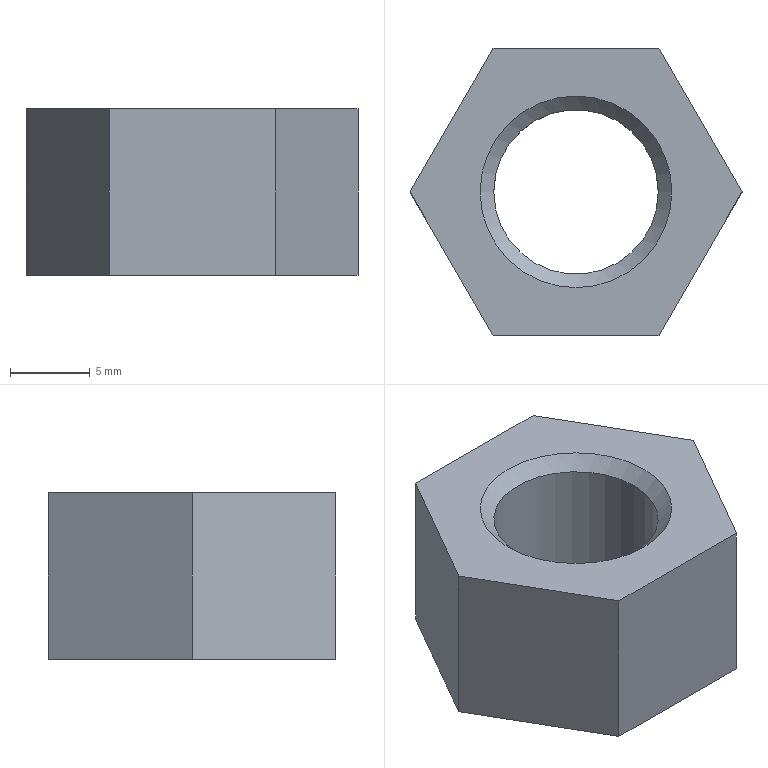Component | NX | 8_2 | 1 solid | 11 faces | box 20.78 x 18 x 10.4 mm | volume 2027 mm3 | plane 8 | cone 2 | cylinder 1 | commonest cylinder face diameters 10.3 x1
STEP:
#1=CARTESIAN_POINT('',(0.,0.,0.));
#2=DIRECTION('',(0.,0.,1.));
#3=DIRECTION('',(1.,0.,0.));
#4=AXIS2_PLACEMENT_3D('',#1,#2,#3);
#5=CARTESIAN_POINT('',(-19.608,30.,47.5));
#6=VERTEX_POINT('',#5);
#7=CARTESIAN_POINT('',(-24.804,39.,47.5));
#8=VERTEX_POINT('',#7);
#9=CARTESIAN_POINT('',(-19.608,30.,47.5));
#10=DIRECTION('',(-0.5,0.866,0.));
#11=VECTOR('',#10,1.);
#12=LINE('',#9,#11);
#13=CARTESIAN_POINT('',(-19.608,30.,57.9));
#14=DIRECTION('',(-0.866,-0.5,0.));
#15=DIRECTION('',(0.5,-0.866,0.));
#16=AXIS2_PLACEMENT_3D('',#13,#14,#15);
#17=PLANE('',#16);
#18=CARTESIAN_POINT('',(0.,-10.4));
#19=DIRECTION('',(-1.,0.));
#20=VECTOR('',#19,1.);
#21=LINE('',#18,#20);
#22=(GEOMETRIC_REPRESENTATION_CONTEXT(2)PARAMETRIC_REPRESENTATION_CONTEXT()REPRESENTATION_CONTEXT('',''));
#23=DEFINITIONAL_REPRESENTATION('',(#21),#22);
#24=PCURVE('',#17,#23);
#25=CARTESIAN_POINT('',(-30.,30.,47.5));
#26=DIRECTION('',(0.,0.,1.));
#27=DIRECTION('',(-1.,-0.00000005,0.));
#28=AXIS2_PLACEMENT_3D('',#25,#26,#27);
#29=PLANE('',#28);
#30=CARTESIAN_POINT('',(-10.392,0.));
#31=DIRECTION('',(0.5,-0.866));
#32=VECTOR('',#31,1.);
#33=LINE('',#30,#32);
#34=(GEOMETRIC_REPRESENTATION_CONTEXT(2)PARAMETRIC_REPRESENTATION_CONTEXT()REPRESENTATION_CONTEXT('',''));
#35=DEFINITIONAL_REPRESENTATION('',(#33),#34);
#36=PCURVE('',#29,#35);
#37=SURFACE_CURVE('',#12,(#24,#36),.PCURVE_S1.);
#38=EDGE_CURVE('',#6,#8,#37,.T.);
#39=ORIENTED_EDGE('',*,*,#38,.T.);
#40=CARTESIAN_POINT('',(-24.804,39.,57.9));
#41=VERTEX_POINT('',#40);
#42=CARTESIAN_POINT('',(-24.804,39.,57.9));
#43=DIRECTION('',(0.,0.,-1.));
#44=VECTOR('',#43,1.);
#45=LINE('',#42,#44);
#46=CARTESIAN_POINT('',(-10.392,0.));
#47=DIRECTION('',(0.,-1.));
#48=VECTOR('',#47,1.);
#49=LINE('',#46,#48);
#50=(GEOMETRIC_REPRESENTATION_CONTEXT(2)PARAMETRIC_REPRESENTATION_CONTEXT()REPRESENTATION_CONTEXT('',''));
#51=DEFINITIONAL_REPRESENTATION('',(#49),#50);
#52=PCURVE('',#17,#51);
#53=CARTESIAN_POINT('',(-24.804,39.,57.9));
#54=DIRECTION('',(0.00000005,-1.,0.));
#55=DIRECTION('',(1.,0.00000005,0.));
#56=AXIS2_PLACEMENT_3D('',#53,#54,#55);
#57=PLANE('',#56);
#58=CARTESIAN_POINT('',(0.,0.));
#59=DIRECTION('',(0.,-1.));
#60=VECTOR('',#59,1.);
#61=LINE('',#58,#60);
#62=(GEOMETRIC_REPRESENTATION_CONTEXT(2)PARAMETRIC_REPRESENTATION_CONTEXT()REPRESENTATION_CONTEXT('',''));
#63=DEFINITIONAL_REPRESENTATION('',(#61),#62);
#64=PCURVE('',#57,#63);
#65=SURFACE_CURVE('',#45,(#52,#64),.PCURVE_S1.);
#66=EDGE_CURVE('',#41,#8,#65,.T.);
#67=ORIENTED_EDGE('',*,*,#66,.F.);
#68=CARTESIAN_POINT('',(-19.608,30.,57.9));
#69=VERTEX_POINT('',#68);
#70=CARTESIAN_POINT('',(-19.608,30.,57.9));
#71=DIRECTION('',(-0.5,0.866,0.));
#72=VECTOR('',#71,1.);
#73=LINE('',#70,#72);
#74=CARTESIAN_POINT('',(0.,0.));
#75=DIRECTION('',(-1.,0.));
#76=VECTOR('',#75,1.);
#77=LINE('',#74,#76);
#78=(GEOMETRIC_REPRESENTATION_CONTEXT(2)PARAMETRIC_REPRESENTATION_CONTEXT()REPRESENTATION_CONTEXT('',''));
#79=DEFINITIONAL_REPRESENTATION('',(#77),#78);
#80=PCURVE('',#17,#79);
#81=CARTESIAN_POINT('',(-30.,30.,57.9));
#82=DIRECTION('',(0.,0.,1.));
#83=DIRECTION('',(-1.,-0.00000005,0.));
#84=AXIS2_PLACEMENT_3D('',#81,#82,#83);
#85=PLANE('',#84);
#86=CARTESIAN_POINT('',(-10.392,0.));
#87=DIRECTION('',(0.5,-0.866));
#88=VECTOR('',#87,1.);
#89=LINE('',#86,#88);
#90=(GEOMETRIC_REPRESENTATION_CONTEXT(2)PARAMETRIC_REPRESENTATION_CONTEXT()REPRESENTATION_CONTEXT('',''));
#91=DEFINITIONAL_REPRESENTATION('',(#89),#90);
#92=PCURVE('',#85,#91);
#93=SURFACE_CURVE('',#73,(#80,#92),.PCURVE_S1.);
#94=EDGE_CURVE('',#69,#41,#93,.T.);
#95=ORIENTED_EDGE('',*,*,#94,.F.);
#96=CARTESIAN_POINT('',(-19.608,30.,57.9));
#97=DIRECTION('',(0.,0.,-1.));
#98=VECTOR('',#97,1.);
#99=LINE('',#96,#98);
#100=CARTESIAN_POINT('',(0.,0.));
#101=DIRECTION('',(0.,-1.));
#102=VECTOR('',#101,1.);
#103=LINE('',#100,#102);
#104=(GEOMETRIC_REPRESENTATION_CONTEXT(2)PARAMETRIC_REPRESENTATION_CONTEXT()REPRESENTATION_CONTEXT('',''));
#105=DEFINITIONAL_REPRESENTATION('',(#103),#104);
#106=PCURVE('',#17,#105);
#107=CARTESIAN_POINT('',(-24.804,21.,57.9));
#108=DIRECTION('',(-0.866,0.5,0.));
#109=DIRECTION('',(-0.5,-0.866,0.));
#110=AXIS2_PLACEMENT_3D('',#107,#108,#109);
#111=PLANE('',#110);
#112=CARTESIAN_POINT('',(-10.392,0.));
#113=DIRECTION('',(0.,-1.));
#114=VECTOR('',#113,1.);
#115=LINE('',#112,#114);
#116=(GEOMETRIC_REPRESENTATION_CONTEXT(2)PARAMETRIC_REPRESENTATION_CONTEXT()REPRESENTATION_CONTEXT('',''));
#117=DEFINITIONAL_REPRESENTATION('',(#115),#116);
#118=PCURVE('',#111,#117);
#119=SURFACE_CURVE('',#99,(#106,#118),.PCURVE_S1.);
#120=EDGE_CURVE('',#69,#6,#119,.T.);
#121=ORIENTED_EDGE('',*,*,#120,.T.);
#122=EDGE_LOOP('',(#39,#67,#95,#121));
#123=FACE_BOUND('',#122,.T.);
#124=ADVANCED_FACE('',(#123),#17,.F.);
#125=CARTESIAN_POINT('',(-35.196,39.,47.5));
#126=VERTEX_POINT('',#125);
#127=CARTESIAN_POINT('',(-24.804,39.,47.5));
#128=DIRECTION('',(-1.,-0.00000005,0.));
#129=VECTOR('',#128,1.);
#130=LINE('',#127,#129);
#131=CARTESIAN_POINT('',(0.,-10.4));
#132=DIRECTION('',(-1.,0.));
#133=VECTOR('',#132,1.);
#134=LINE('',#131,#133);
#135=(GEOMETRIC_REPRESENTATION_CONTEXT(2)PARAMETRIC_REPRESENTATION_CONTEXT()REPRESENTATION_CONTEXT('',''));
#136=DEFINITIONAL_REPRESENTATION('',(#134),#135);
#137=PCURVE('',#57,#136);
#138=CARTESIAN_POINT('',(-5.196,-9.));
#139=DIRECTION('',(1.,-0.));
#140=VECTOR('',#139,1.);
#141=LINE('',#138,#140);
#142=(GEOMETRIC_REPRESENTATION_CONTEXT(2)PARAMETRIC_REPRESENTATION_CONTEXT()REPRESENTATION_CONTEXT('',''));
#143=DEFINITIONAL_REPRESENTATION('',(#141),#142);
#144=PCURVE('',#29,#143);
#145=SURFACE_CURVE('',#130,(#137,#144),.PCURVE_S1.);
#146=EDGE_CURVE('',#8,#126,#145,.T.);
#147=ORIENTED_EDGE('',*,*,#146,.T.);
#148=CARTESIAN_POINT('',(-35.196,39.,57.9));
#149=VERTEX_POINT('',#148);
#150=CARTESIAN_POINT('',(-35.196,39.,57.9));
#151=DIRECTION('',(0.,0.,-1.));
#152=VECTOR('',#151,1.);
#153=LINE('',#150,#152);
#154=CARTESIAN_POINT('',(-10.392,0.));
#155=DIRECTION('',(0.,-1.));
#156=VECTOR('',#155,1.);
#157=LINE('',#154,#156);
#158=(GEOMETRIC_REPRESENTATION_CONTEXT(2)PARAMETRIC_REPRESENTATION_CONTEXT()REPRESENTATION_CONTEXT('',''));
#159=DEFINITIONAL_REPRESENTATION('',(#157),#158);
#160=PCURVE('',#57,#159);
#161=CARTESIAN_POINT('',(-35.196,39.,57.9));
#162=DIRECTION('',(0.866,-0.5,0.));
#163=DIRECTION('',(0.5,0.866,0.));
#164=AXIS2_PLACEMENT_3D('',#161,#162,#163);
#165=PLANE('',#164);
#166=CARTESIAN_POINT('',(0.,0.));
#167=DIRECTION('',(0.,-1.));
#168=VECTOR('',#167,1.);
#169=LINE('',#166,#168);
#170=(GEOMETRIC_REPRESENTATION_CONTEXT(2)PARAMETRIC_REPRESENTATION_CONTEXT()REPRESENTATION_CONTEXT('',''));
#171=DEFINITIONAL_REPRESENTATION('',(#169),#170);
#172=PCURVE('',#165,#171);
#173=SURFACE_CURVE('',#153,(#160,#172),.PCURVE_S1.);
#174=EDGE_CURVE('',#149,#126,#173,.T.);
#175=ORIENTED_EDGE('',*,*,#174,.F.);
#176=CARTESIAN_POINT('',(-24.804,39.,57.9));
#177=DIRECTION('',(-1.,-0.00000005,0.));
#178=VECTOR('',#177,1.);
#179=LINE('',#176,#178);
#180=CARTESIAN_POINT('',(0.,0.));
#181=DIRECTION('',(-1.,0.));
#182=VECTOR('',#181,1.);
#183=LINE('',#180,#182);
#184=(GEOMETRIC_REPRESENTATION_CONTEXT(2)PARAMETRIC_REPRESENTATION_CONTEXT()REPRESENTATION_CONTEXT('',''));
#185=DEFINITIONAL_REPRESENTATION('',(#183),#184);
#186=PCURVE('',#57,#185);
#187=CARTESIAN_POINT('',(-5.196,-9.));
#188=DIRECTION('',(1.,-0.));
#189=VECTOR('',#188,1.);
#190=LINE('',#187,#189);
#191=(GEOMETRIC_REPRESENTATION_CONTEXT(2)PARAMETRIC_REPRESENTATION_CONTEXT()REPRESENTATION_CONTEXT('',''));
#192=DEFINITIONAL_REPRESENTATION('',(#190),#191);
#193=PCURVE('',#85,#192);
#194=SURFACE_CURVE('',#179,(#186,#193),.PCURVE_S1.);
#195=EDGE_CURVE('',#41,#149,#194,.T.);
#196=ORIENTED_EDGE('',*,*,#195,.F.);
#197=ORIENTED_EDGE('',*,*,#66,.T.);
#198=EDGE_LOOP('',(#147,#175,#196,#197));
#199=FACE_BOUND('',#198,.T.);
#200=ADVANCED_FACE('',(#199),#57,.F.);
#201=CARTESIAN_POINT('',(-40.392,30.,47.5));
#202=VERTEX_POINT('',#201);
#203=CARTESIAN_POINT('',(-35.196,39.,47.5));
#204=DIRECTION('',(-0.5,-0.866,0.));
#205=VECTOR('',#204,1.);
#206=LINE('',#203,#205);
#207=CARTESIAN_POINT('',(0.,-10.4));
#208=DIRECTION('',(-1.,0.));
#209=VECTOR('',#208,1.);
#210=LINE('',#207,#209);
#211=(GEOMETRIC_REPRESENTATION_CONTEXT(2)PARAMETRIC_REPRESENTATION_CONTEXT()REPRESENTATION_CONTEXT('',''));
#212=DEFINITIONAL_REPRESENTATION('',(#210),#211);
#213=PCURVE('',#165,#212);
#214=CARTESIAN_POINT('',(5.196,-9.));
#215=DIRECTION('',(0.5,0.866));
#216=VECTOR('',#215,1.);
#217=LINE('',#214,#216);
#218=(GEOMETRIC_REPRESENTATION_CONTEXT(2)PARAMETRIC_REPRESENTATION_CONTEXT()REPRESENTATION_CONTEXT('',''));
#219=DEFINITIONAL_REPRESENTATION('',(#217),#218);
#220=PCURVE('',#29,#219);
#221=SURFACE_CURVE('',#206,(#213,#220),.PCURVE_S1.);
#222=EDGE_CURVE('',#126,#202,#221,.T.);
#223=ORIENTED_EDGE('',*,*,#222,.T.);
#224=CARTESIAN_POINT('',(-40.392,30.,57.9));
#225=VERTEX_POINT('',#224);
#226=CARTESIAN_POINT('',(-40.392,30.,57.9));
#227=DIRECTION('',(0.,0.,-1.));
#228=VECTOR('',#227,1.);
#229=LINE('',#226,#228);
#230=CARTESIAN_POINT('',(-10.392,0.));
#231=DIRECTION('',(0.,-1.));
#232=VECTOR('',#231,1.);
#233=LINE('',#230,#232);
#234=(GEOMETRIC_REPRESENTATION_CONTEXT(2)PARAMETRIC_REPRESENTATION_CONTEXT()REPRESENTATION_CONTEXT('',''));
#235=DEFINITIONAL_REPRESENTATION('',(#233),#234);
#236=PCURVE('',#165,#235);
#237=CARTESIAN_POINT('',(-40.392,30.,57.9));
#238=DIRECTION('',(0.866,0.5,0.));
#239=DIRECTION('',(-0.5,0.866,0.));
#240=AXIS2_PLACEMENT_3D('',#237,#238,#239);
#241=PLANE('',#240);
#242=CARTESIAN_POINT('',(0.,0.));
#243=DIRECTION('',(0.,-1.));
#244=VECTOR('',#243,1.);
#245=LINE('',#242,#244);
#246=(GEOMETRIC_REPRESENTATION_CONTEXT(2)PARAMETRIC_REPRESENTATION_CONTEXT()REPRESENTATION_CONTEXT('',''));
#247=DEFINITIONAL_REPRESENTATION('',(#245),#246);
#248=PCURVE('',#241,#247);
#249=SURFACE_CURVE('',#229,(#236,#248),.PCURVE_S1.);
#250=EDGE_CURVE('',#225,#202,#249,.T.);
#251=ORIENTED_EDGE('',*,*,#250,.F.);
#252=CARTESIAN_POINT('',(-35.196,39.,57.9));
#253=DIRECTION('',(-0.5,-0.866,0.));
#254=VECTOR('',#253,1.);
#255=LINE('',#252,#254);
#256=CARTESIAN_POINT('',(0.,0.));
#257=DIRECTION('',(-1.,0.));
#258=VECTOR('',#257,1.);
#259=LINE('',#256,#258);
#260=(GEOMETRIC_REPRESENTATION_CONTEXT(2)PARAMETRIC_REPRESENTATION_CONTEXT()REPRESENTATION_CONTEXT('',''));
#261=DEFINITIONAL_REPRESENTATION('',(#259),#260);
#262=PCURVE('',#165,#261);
#263=CARTESIAN_POINT('',(5.196,-9.));
#264=DIRECTION('',(0.5,0.866));
#265=VECTOR('',#264,1.);
#266=LINE('',#263,#265);
#267=(GEOMETRIC_REPRESENTATION_CONTEXT(2)PARAMETRIC_REPRESENTATION_CONTEXT()REPRESENTATION_CONTEXT('',''));
#268=DEFINITIONAL_REPRESENTATION('',(#266),#267);
#269=PCURVE('',#85,#268);
#270=SURFACE_CURVE('',#255,(#262,#269),.PCURVE_S1.);
#271=EDGE_CURVE('',#149,#225,#270,.T.);
#272=ORIENTED_EDGE('',*,*,#271,.F.);
#273=ORIENTED_EDGE('',*,*,#174,.T.);
#274=EDGE_LOOP('',(#223,#251,#272,#273));
#275=FACE_BOUND('',#274,.T.);
#276=ADVANCED_FACE('',(#275),#165,.F.);
#277=CARTESIAN_POINT('',(-35.196,21.,47.5));
#278=VERTEX_POINT('',#277);
#279=CARTESIAN_POINT('',(-40.392,30.,47.5));
#280=DIRECTION('',(0.5,-0.866,0.));
#281=VECTOR('',#280,1.);
#282=LINE('',#279,#281);
#283=CARTESIAN_POINT('',(0.,-10.4));
#284=DIRECTION('',(-1.,0.));
#285=VECTOR('',#284,1.);
#286=LINE('',#283,#285);
#287=(GEOMETRIC_REPRESENTATION_CONTEXT(2)PARAMETRIC_REPRESENTATION_CONTEXT()REPRESENTATION_CONTEXT('',''));
#288=DEFINITIONAL_REPRESENTATION('',(#286),#287);
#289=PCURVE('',#241,#288);
#290=CARTESIAN_POINT('',(10.392,-0.));
#291=DIRECTION('',(-0.5,0.866));
#292=VECTOR('',#291,1.);
#293=LINE('',#290,#292);
#294=(GEOMETRIC_REPRESENTATION_CONTEXT(2)PARAMETRIC_REPRESENTATION_CONTEXT()REPRESENTATION_CONTEXT('',''));
#295=DEFINITIONAL_REPRESENTATION('',(#293),#294);
#296=PCURVE('',#29,#295);
#297=SURFACE_CURVE('',#282,(#289,#296),.PCURVE_S1.);
#298=EDGE_CURVE('',#202,#278,#297,.T.);
#299=ORIENTED_EDGE('',*,*,#298,.T.);
#300=CARTESIAN_POINT('',(-35.196,21.,57.9));
#301=VERTEX_POINT('',#300);
#302=CARTESIAN_POINT('',(-35.196,21.,57.9));
#303=DIRECTION('',(0.,0.,-1.));
#304=VECTOR('',#303,1.);
#305=LINE('',#302,#304);
#306=CARTESIAN_POINT('',(-10.392,0.));
#307=DIRECTION('',(0.,-1.));
#308=VECTOR('',#307,1.);
#309=LINE('',#306,#308);
#310=(GEOMETRIC_REPRESENTATION_CONTEXT(2)PARAMETRIC_REPRESENTATION_CONTEXT()REPRESENTATION_CONTEXT('',''));
#311=DEFINITIONAL_REPRESENTATION('',(#309),#310);
#312=PCURVE('',#241,#311);
#313=CARTESIAN_POINT('',(-35.196,21.,57.9));
#314=DIRECTION('',(-0.00000005,1.,0.));
#315=DIRECTION('',(-1.,-0.00000005,0.));
#316=AXIS2_PLACEMENT_3D('',#313,#314,#315);
#317=PLANE('',#316);
#318=CARTESIAN_POINT('',(0.,0.));
#319=DIRECTION('',(0.,-1.));
#320=VECTOR('',#319,1.);
#321=LINE('',#318,#320);
#322=(GEOMETRIC_REPRESENTATION_CONTEXT(2)PARAMETRIC_REPRESENTATION_CONTEXT()REPRESENTATION_CONTEXT('',''));
#323=DEFINITIONAL_REPRESENTATION('',(#321),#322);
#324=PCURVE('',#317,#323);
#325=SURFACE_CURVE('',#305,(#312,#324),.PCURVE_S1.);
#326=EDGE_CURVE('',#301,#278,#325,.T.);
#327=ORIENTED_EDGE('',*,*,#326,.F.);
#328=CARTESIAN_POINT('',(-40.392,30.,57.9));
#329=DIRECTION('',(0.5,-0.866,0.));
#330=VECTOR('',#329,1.);
#331=LINE('',#328,#330);
#332=CARTESIAN_POINT('',(0.,0.));
#333=DIRECTION('',(-1.,0.));
#334=VECTOR('',#333,1.);
#335=LINE('',#332,#334);
#336=(GEOMETRIC_REPRESENTATION_CONTEXT(2)PARAMETRIC_REPRESENTATION_CONTEXT()REPRESENTATION_CONTEXT('',''));
#337=DEFINITIONAL_REPRESENTATION('',(#335),#336);
#338=PCURVE('',#241,#337);
#339=CARTESIAN_POINT('',(10.392,-0.));
#340=DIRECTION('',(-0.5,0.866));
#341=VECTOR('',#340,1.);
#342=LINE('',#339,#341);
#343=(GEOMETRIC_REPRESENTATION_CONTEXT(2)PARAMETRIC_REPRESENTATION_CONTEXT()REPRESENTATION_CONTEXT('',''));
#344=DEFINITIONAL_REPRESENTATION('',(#342),#343);
#345=PCURVE('',#85,#344);
#346=SURFACE_CURVE('',#331,(#338,#345),.PCURVE_S1.);
#347=EDGE_CURVE('',#225,#301,#346,.T.);
#348=ORIENTED_EDGE('',*,*,#347,.F.);
#349=ORIENTED_EDGE('',*,*,#250,.T.);
#350=EDGE_LOOP('',(#299,#327,#348,#349));
#351=FACE_BOUND('',#350,.T.);
#352=ADVANCED_FACE('',(#351),#241,.F.);
#353=CARTESIAN_POINT('',(-24.804,21.,47.5));
#354=VERTEX_POINT('',#353);
#355=CARTESIAN_POINT('',(-35.196,21.,47.5));
#356=DIRECTION('',(1.,0.00000005,0.));
#357=VECTOR('',#356,1.);
#358=LINE('',#355,#357);
#359=CARTESIAN_POINT('',(0.,-10.4));
#360=DIRECTION('',(-1.,0.));
#361=VECTOR('',#360,1.);
#362=LINE('',#359,#361);
#363=(GEOMETRIC_REPRESENTATION_CONTEXT(2)PARAMETRIC_REPRESENTATION_CONTEXT()REPRESENTATION_CONTEXT('',''));
#364=DEFINITIONAL_REPRESENTATION('',(#362),#363);
#365=PCURVE('',#317,#364);
#366=CARTESIAN_POINT('',(5.196,9.));
#367=DIRECTION('',(-1.,0.));
#368=VECTOR('',#367,1.);
#369=LINE('',#366,#368);
#370=(GEOMETRIC_REPRESENTATION_CONTEXT(2)PARAMETRIC_REPRESENTATION_CONTEXT()REPRESENTATION_CONTEXT('',''));
#371=DEFINITIONAL_REPRESENTATION('',(#369),#370);
#372=PCURVE('',#29,#371);
#373=SURFACE_CURVE('',#358,(#365,#372),.PCURVE_S1.);
#374=EDGE_CURVE('',#278,#354,#373,.T.);
#375=ORIENTED_EDGE('',*,*,#374,.T.);
#376=CARTESIAN_POINT('',(-24.804,21.,57.9));
#377=VERTEX_POINT('',#376);
#378=CARTESIAN_POINT('',(-24.804,21.,57.9));
#379=DIRECTION('',(0.,0.,-1.));
#380=VECTOR('',#379,1.);
#381=LINE('',#378,#380);
#382=CARTESIAN_POINT('',(-10.392,0.));
#383=DIRECTION('',(0.,-1.));
#384=VECTOR('',#383,1.);
#385=LINE('',#382,#384);
#386=(GEOMETRIC_REPRESENTATION_CONTEXT(2)PARAMETRIC_REPRESENTATION_CONTEXT()REPRESENTATION_CONTEXT('',''));
#387=DEFINITIONAL_REPRESENTATION('',(#385),#386);
#388=PCURVE('',#317,#387);
#389=CARTESIAN_POINT('',(0.,0.));
#390=DIRECTION('',(0.,-1.));
#391=VECTOR('',#390,1.);
#392=LINE('',#389,#391);
#393=(GEOMETRIC_REPRESENTATION_CONTEXT(2)PARAMETRIC_REPRESENTATION_CONTEXT()REPRESENTATION_CONTEXT('',''));
#394=DEFINITIONAL_REPRESENTATION('',(#392),#393);
#395=PCURVE('',#111,#394);
#396=SURFACE_CURVE('',#381,(#388,#395),.PCURVE_S1.);
#397=EDGE_CURVE('',#377,#354,#396,.T.);
#398=ORIENTED_EDGE('',*,*,#397,.F.);
#399=CARTESIAN_POINT('',(-35.196,21.,57.9));
#400=DIRECTION('',(1.,0.00000005,0.));
#401=VECTOR('',#400,1.);
#402=LINE('',#399,#401);
#403=CARTESIAN_POINT('',(0.,0.));
#404=DIRECTION('',(-1.,0.));
#405=VECTOR('',#404,1.);
#406=LINE('',#403,#405);
#407=(GEOMETRIC_REPRESENTATION_CONTEXT(2)PARAMETRIC_REPRESENTATION_CONTEXT()REPRESENTATION_CONTEXT('',''));
#408=DEFINITIONAL_REPRESENTATION('',(#406),#407);
#409=PCURVE('',#317,#408);
#410=CARTESIAN_POINT('',(5.196,9.));
#411=DIRECTION('',(-1.,0.));
#412=VECTOR('',#411,1.);
#413=LINE('',#410,#412);
#414=(GEOMETRIC_REPRESENTATION_CONTEXT(2)PARAMETRIC_REPRESENTATION_CONTEXT()REPRESENTATION_CONTEXT('',''));
#415=DEFINITIONAL_REPRESENTATION('',(#413),#414);
#416=PCURVE('',#85,#415);
#417=SURFACE_CURVE('',#402,(#409,#416),.PCURVE_S1.);
#418=EDGE_CURVE('',#301,#377,#417,.T.);
#419=ORIENTED_EDGE('',*,*,#418,.F.);
#420=ORIENTED_EDGE('',*,*,#326,.T.);
#421=EDGE_LOOP('',(#375,#398,#419,#420));
#422=FACE_BOUND('',#421,.T.);
#423=ADVANCED_FACE('',(#422),#317,.F.);
#424=CARTESIAN_POINT('',(-24.804,21.,47.5));
#425=DIRECTION('',(0.5,0.866,0.));
#426=VECTOR('',#425,1.);
#427=LINE('',#424,#426);
#428=CARTESIAN_POINT('',(0.,-10.4));
#429=DIRECTION('',(-1.,0.));
#430=VECTOR('',#429,1.);
#431=LINE('',#428,#430);
#432=(GEOMETRIC_REPRESENTATION_CONTEXT(2)PARAMETRIC_REPRESENTATION_CONTEXT()REPRESENTATION_CONTEXT('',''));
#433=DEFINITIONAL_REPRESENTATION('',(#431),#432);
#434=PCURVE('',#111,#433);
#435=CARTESIAN_POINT('',(-5.196,9.));
#436=DIRECTION('',(-0.5,-0.866));
#437=VECTOR('',#436,1.);
#438=LINE('',#435,#437);
#439=(GEOMETRIC_REPRESENTATION_CONTEXT(2)PARAMETRIC_REPRESENTATION_CONTEXT()REPRESENTATION_CONTEXT('',''));
#440=DEFINITIONAL_REPRESENTATION('',(#438),#439);
#441=PCURVE('',#29,#440);
#442=SURFACE_CURVE('',#427,(#434,#441),.PCURVE_S1.);
#443=EDGE_CURVE('',#354,#6,#442,.T.);
#444=ORIENTED_EDGE('',*,*,#443,.T.);
#445=ORIENTED_EDGE('',*,*,#120,.F.);
#446=CARTESIAN_POINT('',(-24.804,21.,57.9));
#447=DIRECTION('',(0.5,0.866,0.));
#448=VECTOR('',#447,1.);
#449=LINE('',#446,#448);
#450=CARTESIAN_POINT('',(0.,0.));
#451=DIRECTION('',(-1.,0.));
#452=VECTOR('',#451,1.);
#453=LINE('',#450,#452);
#454=(GEOMETRIC_REPRESENTATION_CONTEXT(2)PARAMETRIC_REPRESENTATION_CONTEXT()REPRESENTATION_CONTEXT('',''));
#455=DEFINITIONAL_REPRESENTATION('',(#453),#454);
#456=PCURVE('',#111,#455);
#457=CARTESIAN_POINT('',(-5.196,9.));
#458=DIRECTION('',(-0.5,-0.866));
#459=VECTOR('',#458,1.);
#460=LINE('',#457,#459);
#461=(GEOMETRIC_REPRESENTATION_CONTEXT(2)PARAMETRIC_REPRESENTATION_CONTEXT()REPRESENTATION_CONTEXT('',''));
#462=DEFINITIONAL_REPRESENTATION('',(#460),#461);
#463=PCURVE('',#85,#462);
#464=SURFACE_CURVE('',#449,(#456,#463),.PCURVE_S1.);
#465=EDGE_CURVE('',#377,#69,#464,.T.);
#466=ORIENTED_EDGE('',*,*,#465,.F.);
#467=ORIENTED_EDGE('',*,*,#397,.T.);
#468=EDGE_LOOP('',(#444,#445,#466,#467));
#469=FACE_BOUND('',#468,.T.);
#470=ADVANCED_FACE('',(#469),#111,.F.);
#471=CARTESIAN_POINT('',(-36.,30.,57.9));
#472=VERTEX_POINT('',#471);
#473=CARTESIAN_POINT('',(-30.,30.,57.9));
#474=DIRECTION('',(0.,0.,-1.));
#475=DIRECTION('',(-1.,-0.00000005,0.));
#476=AXIS2_PLACEMENT_3D('',#473,#474,#475);
#477=CIRCLE('',#476,6.);
#478=CARTESIAN_POINT('',(6.,-0.));
#479=CARTESIAN_POINT('',(6.,-10.392));
#480=CARTESIAN_POINT('',(-3.,-5.196));
#481=CARTESIAN_POINT('',(-12.,0.));
#482=CARTESIAN_POINT('',(-3.,5.196));
#483=CARTESIAN_POINT('',(6.,10.392));
#484=CARTESIAN_POINT('',(6.,-0.));
#485=(BOUNDED_CURVE()B_SPLINE_CURVE(2,(#478,#479,#480,#481,#482,#483,#484),.UNSPECIFIED.,.T.,.F.)B_SPLINE_CURVE_WITH_KNOTS((1,2,2,2,2,1),(-2.094,0.,2.094,4.189,6.283,8.378),.UNSPECIFIED.)CURVE()GEOMETRIC_REPRESENTATION_ITEM()RATIONAL_B_SPLINE_CURVE((1.,0.5,1.,0.5,1.,0.5,1.))REPRESENTATION_ITEM(''));
#486=(GEOMETRIC_REPRESENTATION_CONTEXT(2)PARAMETRIC_REPRESENTATION_CONTEXT()REPRESENTATION_CONTEXT('',''));
#487=DEFINITIONAL_REPRESENTATION('',(#485),#486);
#488=PCURVE('',#85,#487);
#489=CARTESIAN_POINT('',(-30.,30.,57.05));
#490=DIRECTION('',(0.,0.,1.));
#491=DIRECTION('',(-1.,-0.00000005,0.));
#492=AXIS2_PLACEMENT_3D('',#489,#490,#491);
#493=CONICAL_SURFACE('',#492,5.15,0.7854);
#494=CARTESIAN_POINT('',(6.283,0.85));
#495=DIRECTION('',(-1.,0.));
#496=VECTOR('',#495,1.);
#497=LINE('',#494,#496);
#498=(GEOMETRIC_REPRESENTATION_CONTEXT(2)PARAMETRIC_REPRESENTATION_CONTEXT()REPRESENTATION_CONTEXT('',''));
#499=DEFINITIONAL_REPRESENTATION('',(#497),#498);
#500=PCURVE('',#493,#499);
#501=SURFACE_CURVE('',#477,(#488,#500),.PCURVE_S1.);
#502=EDGE_CURVE('',#472,#472,#501,.T.);
#503=ORIENTED_EDGE('',*,*,#502,.T.);
#504=EDGE_LOOP('',(#503));
#505=FACE_BOUND('',#504,.T.);
#506=ORIENTED_EDGE('',*,*,#94,.T.);
#507=ORIENTED_EDGE('',*,*,#195,.T.);
#508=ORIENTED_EDGE('',*,*,#271,.T.);
#509=ORIENTED_EDGE('',*,*,#347,.T.);
#510=ORIENTED_EDGE('',*,*,#418,.T.);
#511=ORIENTED_EDGE('',*,*,#465,.T.);
#512=EDGE_LOOP('',(#506,#507,#508,#509,#510,#511));
#513=FACE_BOUND('',#512,.T.);
#514=ADVANCED_FACE('',(#505,#513),#85,.T.);
#515=CARTESIAN_POINT('',(-36.,30.,47.5));
#516=VERTEX_POINT('',#515);
#517=CARTESIAN_POINT('',(-30.,30.,47.5));
#518=DIRECTION('',(0.,0.,1.));
#519=DIRECTION('',(-1.,-0.00000005,0.));
#520=AXIS2_PLACEMENT_3D('',#517,#518,#519);
#521=CIRCLE('',#520,6.);
#522=CARTESIAN_POINT('',(0.,0.));
#523=DIRECTION('',(1.,-0.));
#524=AXIS2_PLACEMENT_2D('',#522,#523);
#525=CIRCLE('',#524,6.);
#526=(GEOMETRIC_REPRESENTATION_CONTEXT(2)PARAMETRIC_REPRESENTATION_CONTEXT()REPRESENTATION_CONTEXT('',''));
#527=DEFINITIONAL_REPRESENTATION('',(#525),#526);
#528=PCURVE('',#29,#527);
#529=CARTESIAN_POINT('',(-30.,30.,47.5));
#530=DIRECTION('',(0.,0.,-1.));
#531=DIRECTION('',(1.,0.00000005,0.));
#532=AXIS2_PLACEMENT_3D('',#529,#530,#531);
#533=CONICAL_SURFACE('',#532,6.,0.7854);
#534=CARTESIAN_POINT('',(9.425,-0.));
#535=DIRECTION('',(-1.,0.));
#536=VECTOR('',#535,1.);
#537=LINE('',#534,#536);
#538=(GEOMETRIC_REPRESENTATION_CONTEXT(2)PARAMETRIC_REPRESENTATION_CONTEXT()REPRESENTATION_CONTEXT('',''));
#539=DEFINITIONAL_REPRESENTATION('',(#537),#538);
#540=PCURVE('',#533,#539);
#541=SURFACE_CURVE('',#521,(#528,#540),.PCURVE_S1.);
#542=EDGE_CURVE('',#516,#516,#541,.T.);
#543=ORIENTED_EDGE('',*,*,#542,.T.);
#544=EDGE_LOOP('',(#543));
#545=FACE_BOUND('',#544,.T.);
#546=ORIENTED_EDGE('',*,*,#38,.F.);
#547=ORIENTED_EDGE('',*,*,#443,.F.);
#548=ORIENTED_EDGE('',*,*,#374,.F.);
#549=ORIENTED_EDGE('',*,*,#298,.F.);
#550=ORIENTED_EDGE('',*,*,#222,.F.);
#551=ORIENTED_EDGE('',*,*,#146,.F.);
#552=EDGE_LOOP('',(#546,#547,#548,#549,#550,#551));
#553=FACE_BOUND('',#552,.T.);
#554=ADVANCED_FACE('',(#545,#553),#29,.F.);
#555=CARTESIAN_POINT('',(-35.15,30.,57.05));
#556=VERTEX_POINT('',#555);
#557=CARTESIAN_POINT('',(-30.,30.,57.05));
#558=DIRECTION('',(0.,0.,1.));
#559=DIRECTION('',(-1.,-0.00000005,0.));
#560=AXIS2_PLACEMENT_3D('',#557,#558,#559);
#561=CIRCLE('',#560,5.15);
#562=CARTESIAN_POINT('',(-30.,30.,47.5));
#563=DIRECTION('',(0.,0.,1.));
#564=DIRECTION('',(-1.,-0.00000005,0.));
#565=AXIS2_PLACEMENT_3D('',#562,#563,#564);
#566=CYLINDRICAL_SURFACE('',#565,5.15);
#567=CARTESIAN_POINT('',(0.,9.55));
#568=DIRECTION('',(1.,0.));
#569=VECTOR('',#568,1.);
#570=LINE('',#567,#569);
#571=(GEOMETRIC_REPRESENTATION_CONTEXT(2)PARAMETRIC_REPRESENTATION_CONTEXT()REPRESENTATION_CONTEXT('',''));
#572=DEFINITIONAL_REPRESENTATION('',(#570),#571);
#573=PCURVE('',#566,#572);
#574=CARTESIAN_POINT('',(0.,0.));
#575=DIRECTION('',(1.,0.));
#576=VECTOR('',#575,1.);
#577=LINE('',#574,#576);
#578=(GEOMETRIC_REPRESENTATION_CONTEXT(2)PARAMETRIC_REPRESENTATION_CONTEXT()REPRESENTATION_CONTEXT('',''));
#579=DEFINITIONAL_REPRESENTATION('',(#577),#578);
#580=PCURVE('',#493,#579);
#581=SURFACE_CURVE('',#561,(#573,#580),.PCURVE_S1.);
#582=EDGE_CURVE('',#556,#556,#581,.T.);
#583=ORIENTED_EDGE('',*,*,#582,.F.);
#584=CARTESIAN_POINT('',(-35.15,30.,48.35));
#585=VERTEX_POINT('',#584);
#586=CARTESIAN_POINT('',(-35.15,30.,48.35));
#587=CARTESIAN_POINT('',(-35.15,30.,57.05));
#588=B_SPLINE_CURVE_WITH_KNOTS('',1,(#586,#587),.UNSPECIFIED.,.F.,.F.,(2,2),(0.85,9.55),.PIECEWISE_BEZIER_KNOTS.);
#589=CARTESIAN_POINT('',(0.,0.));
#590=DIRECTION('',(0.,1.));
#591=VECTOR('',#590,1.);
#592=LINE('',#589,#591);
#593=(GEOMETRIC_REPRESENTATION_CONTEXT(2)PARAMETRIC_REPRESENTATION_CONTEXT()REPRESENTATION_CONTEXT('',''));
#594=DEFINITIONAL_REPRESENTATION('',(#592),#593);
#595=PCURVE('',#566,#594);
#596=CARTESIAN_POINT('',(6.283,0.));
#597=DIRECTION('',(0.,1.));
#598=VECTOR('',#597,1.);
#599=LINE('',#596,#598);
#600=(GEOMETRIC_REPRESENTATION_CONTEXT(2)PARAMETRIC_REPRESENTATION_CONTEXT()REPRESENTATION_CONTEXT('',''));
#601=DEFINITIONAL_REPRESENTATION('',(#599),#600);
#602=PCURVE('',#566,#601);
#603=SEAM_CURVE('',#588,(#595,#602),.PCURVE_S1.);
#604=EDGE_CURVE('',#585,#556,#603,.T.);
#605=ORIENTED_EDGE('',*,*,#604,.F.);
#606=CARTESIAN_POINT('',(-30.,30.,48.35));
#607=DIRECTION('',(0.,0.,-1.));
#608=DIRECTION('',(-1.,-0.00000005,0.));
#609=AXIS2_PLACEMENT_3D('',#606,#607,#608);
#610=CIRCLE('',#609,5.15);
#611=CARTESIAN_POINT('',(6.283,0.85));
#612=DIRECTION('',(-1.,0.));
#613=VECTOR('',#612,1.);
#614=LINE('',#611,#613);
#615=(GEOMETRIC_REPRESENTATION_CONTEXT(2)PARAMETRIC_REPRESENTATION_CONTEXT()REPRESENTATION_CONTEXT('',''));
#616=DEFINITIONAL_REPRESENTATION('',(#614),#615);
#617=PCURVE('',#566,#616);
#618=CARTESIAN_POINT('',(3.142,-0.85));
#619=DIRECTION('',(1.,0.));
#620=VECTOR('',#619,1.);
#621=LINE('',#618,#620);
#622=(GEOMETRIC_REPRESENTATION_CONTEXT(2)PARAMETRIC_REPRESENTATION_CONTEXT()REPRESENTATION_CONTEXT('',''));
#623=DEFINITIONAL_REPRESENTATION('',(#621),#622);
#624=PCURVE('',#533,#623);
#625=SURFACE_CURVE('',#610,(#617,#624),.PCURVE_S1.);
#626=EDGE_CURVE('',#585,#585,#625,.T.);
#627=ORIENTED_EDGE('',*,*,#626,.F.);
#628=ORIENTED_EDGE('',*,*,#604,.T.);
#629=EDGE_LOOP('',(#583,#605,#627,#628));
#630=FACE_BOUND('',#629,.F.);
#631=ADVANCED_FACE('',(#630),#566,.F.);
#632=ORIENTED_EDGE('',*,*,#626,.T.);
#633=CARTESIAN_POINT('',(-35.15,30.,48.35));
#634=CARTESIAN_POINT('',(-36.,30.,47.5));
#635=B_SPLINE_CURVE_WITH_KNOTS('',1,(#633,#634),.UNSPECIFIED.,.F.,.F.,(2,2),(-1.202,-0.),.PIECEWISE_BEZIER_KNOTS.);
#636=CARTESIAN_POINT('',(9.425,0.));
#637=DIRECTION('',(0.,1.));
#638=VECTOR('',#637,1.);
#639=LINE('',#636,#638);
#640=(GEOMETRIC_REPRESENTATION_CONTEXT(2)PARAMETRIC_REPRESENTATION_CONTEXT()REPRESENTATION_CONTEXT('',''));
#641=DEFINITIONAL_REPRESENTATION('',(#639),#640);
#642=PCURVE('',#533,#641);
#643=CARTESIAN_POINT('',(3.142,0.));
#644=DIRECTION('',(0.,1.));
#645=VECTOR('',#644,1.);
#646=LINE('',#643,#645);
#647=(GEOMETRIC_REPRESENTATION_CONTEXT(2)PARAMETRIC_REPRESENTATION_CONTEXT()REPRESENTATION_CONTEXT('',''));
#648=DEFINITIONAL_REPRESENTATION('',(#646),#647);
#649=PCURVE('',#533,#648);
#650=SEAM_CURVE('',#635,(#642,#649),.PCURVE_S1.);
#651=EDGE_CURVE('',#585,#516,#650,.T.);
#652=ORIENTED_EDGE('',*,*,#651,.T.);
#653=ORIENTED_EDGE('',*,*,#542,.T.);
#654=ORIENTED_EDGE('',*,*,#651,.F.);
#655=EDGE_LOOP('',(#632,#652,#653,#654));
#656=FACE_BOUND('',#655,.F.);
#657=ADVANCED_FACE('',(#656),#533,.F.);
#658=ORIENTED_EDGE('',*,*,#502,.T.);
#659=CARTESIAN_POINT('',(-35.15,30.,57.05));
#660=CARTESIAN_POINT('',(-36.,30.,57.9));
#661=B_SPLINE_CURVE_WITH_KNOTS('',1,(#659,#660),.UNSPECIFIED.,.F.,.F.,(2,2),(0.,1.202),.PIECEWISE_BEZIER_KNOTS.);
#662=CARTESIAN_POINT('',(0.,0.));
#663=DIRECTION('',(0.,1.));
#664=VECTOR('',#663,1.);
#665=LINE('',#662,#664);
#666=(GEOMETRIC_REPRESENTATION_CONTEXT(2)PARAMETRIC_REPRESENTATION_CONTEXT()REPRESENTATION_CONTEXT('',''));
#667=DEFINITIONAL_REPRESENTATION('',(#665),#666);
#668=PCURVE('',#493,#667);
#669=CARTESIAN_POINT('',(6.283,0.));
#670=DIRECTION('',(0.,1.));
#671=VECTOR('',#670,1.);
#672=LINE('',#669,#671);
#673=(GEOMETRIC_REPRESENTATION_CONTEXT(2)PARAMETRIC_REPRESENTATION_CONTEXT()REPRESENTATION_CONTEXT('',''));
#674=DEFINITIONAL_REPRESENTATION('',(#672),#673);
#675=PCURVE('',#493,#674);
#676=SEAM_CURVE('',#661,(#668,#675),.PCURVE_S1.);
#677=EDGE_CURVE('',#556,#472,#676,.T.);
#678=ORIENTED_EDGE('',*,*,#677,.F.);
#679=ORIENTED_EDGE('',*,*,#582,.T.);
#680=ORIENTED_EDGE('',*,*,#677,.T.);
#681=EDGE_LOOP('',(#658,#678,#679,#680));
#682=FACE_BOUND('',#681,.F.);
#683=ADVANCED_FACE('',(#682),#493,.F.);
#684=CLOSED_SHELL('',(#124,#200,#276,#352,#423,#470,#514,#554,#631,#657,#683));
#685=MANIFOLD_SOLID_BREP('',#684);
#686=(LENGTH_UNIT()NAMED_UNIT(*)SI_UNIT(.MILLI.,.METRE.));
#687=UNCERTAINTY_MEASURE_WITH_UNIT(LENGTH_MEASURE(0.000002),#686,'','');
#688=(NAMED_UNIT(*)PLANE_ANGLE_UNIT()SI_UNIT($,.RADIAN.));
#689=(NAMED_UNIT(*)SI_UNIT($,.STERADIAN.)SOLID_ANGLE_UNIT());
#690=(GEOMETRIC_REPRESENTATION_CONTEXT(3)GLOBAL_UNCERTAINTY_ASSIGNED_CONTEXT((#687))GLOBAL_UNIT_ASSIGNED_CONTEXT((#686,#688,#689))REPRESENTATION_CONTEXT('',''));
#691=ADVANCED_BREP_SHAPE_REPRESENTATION('',(#4,#685),#690);